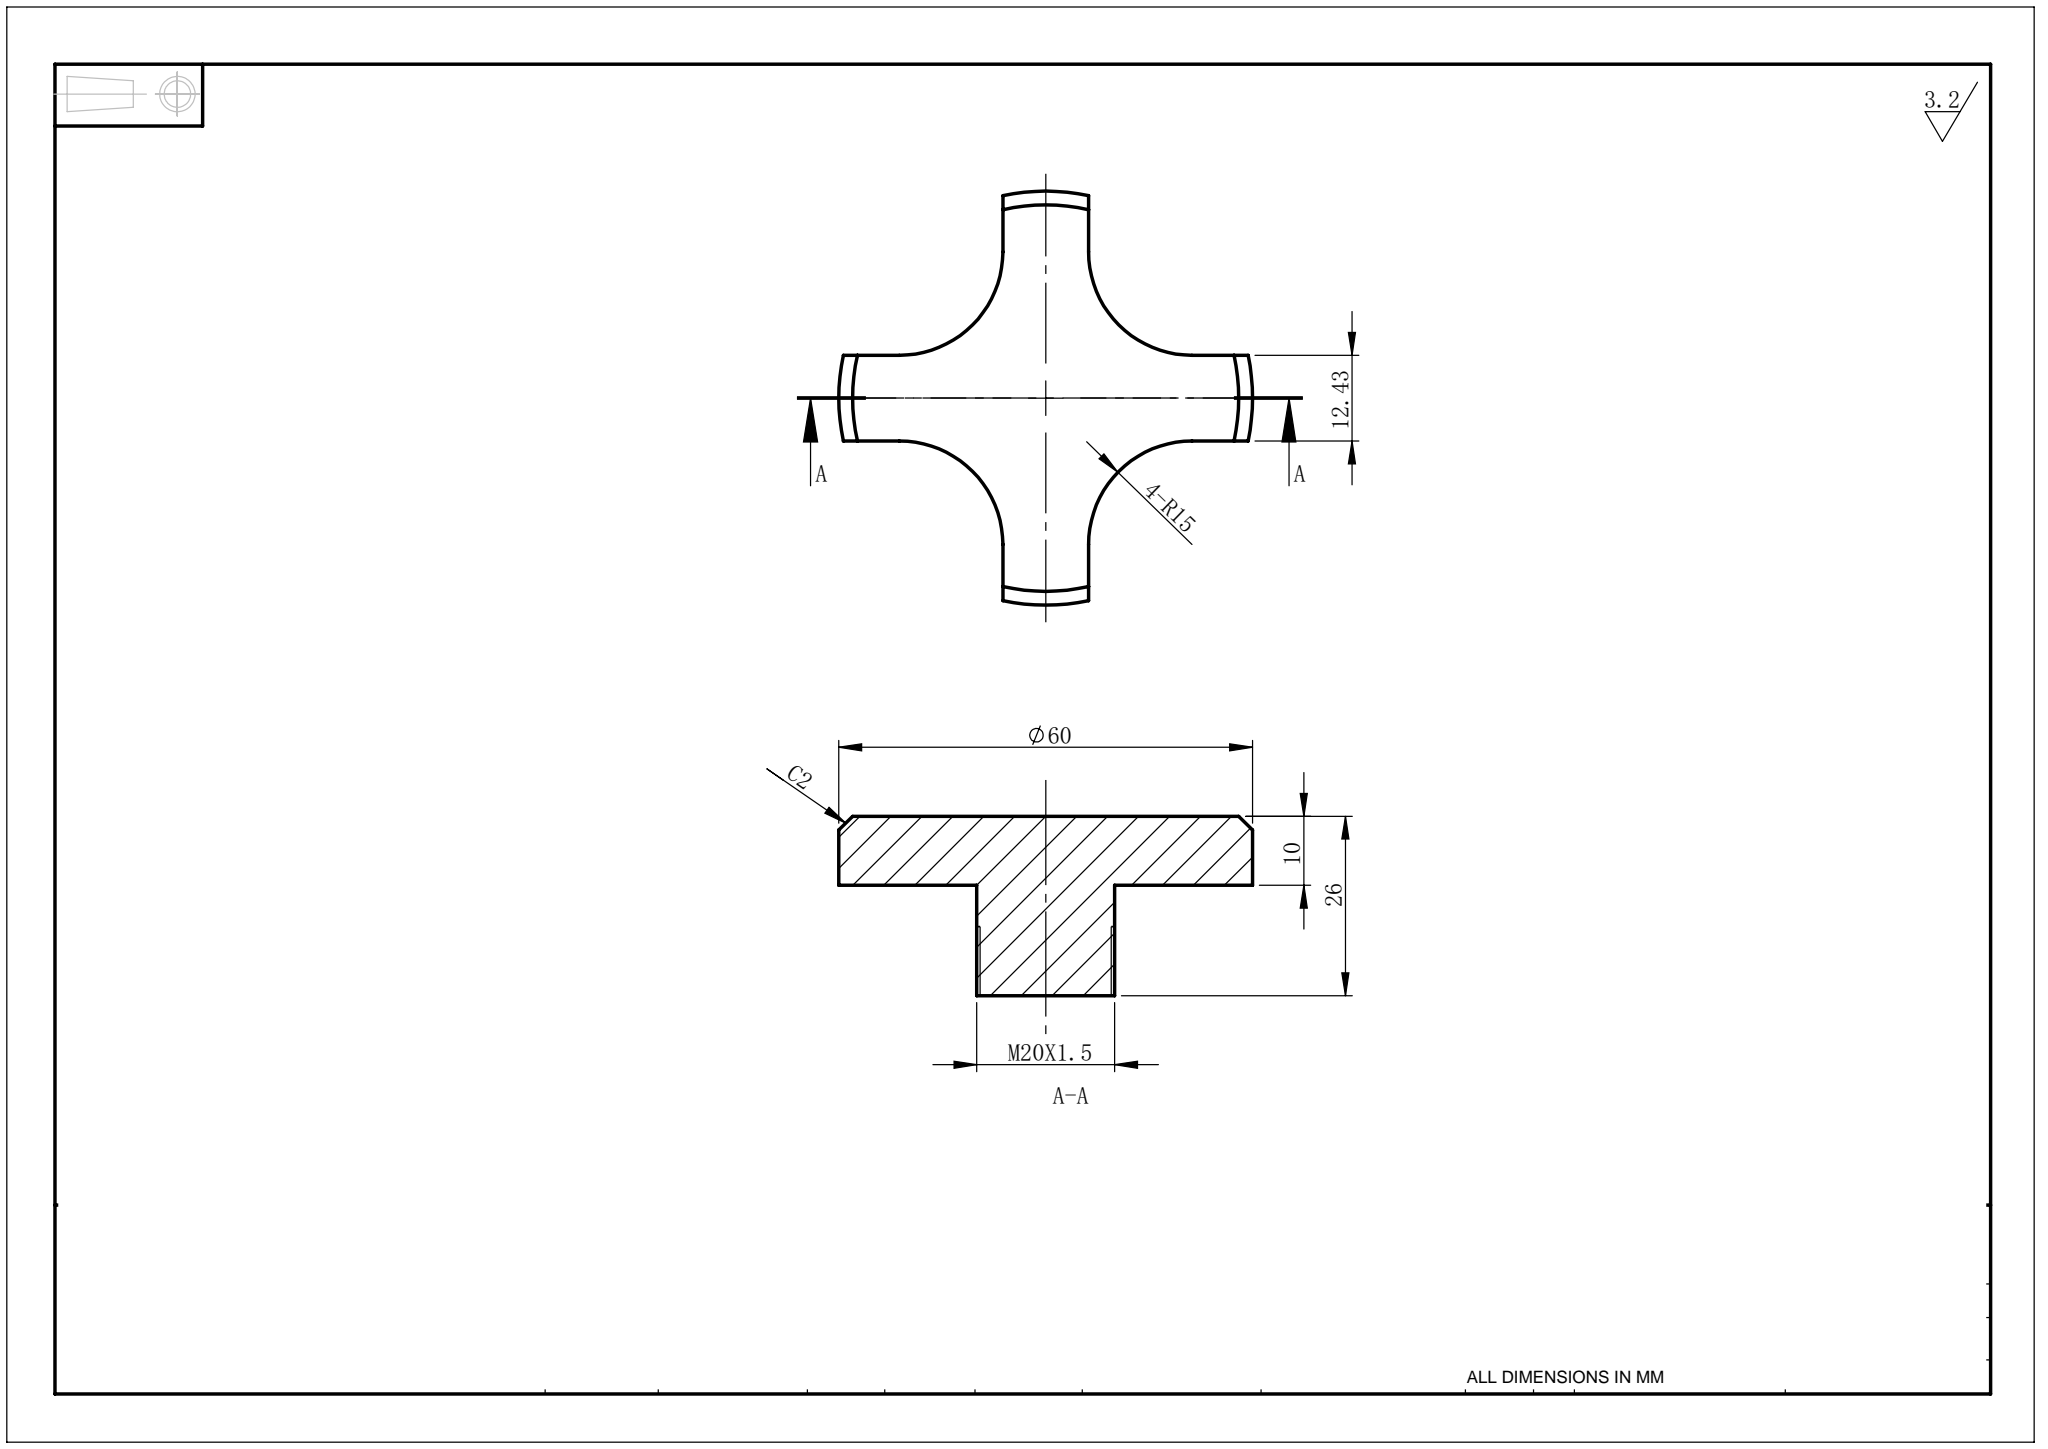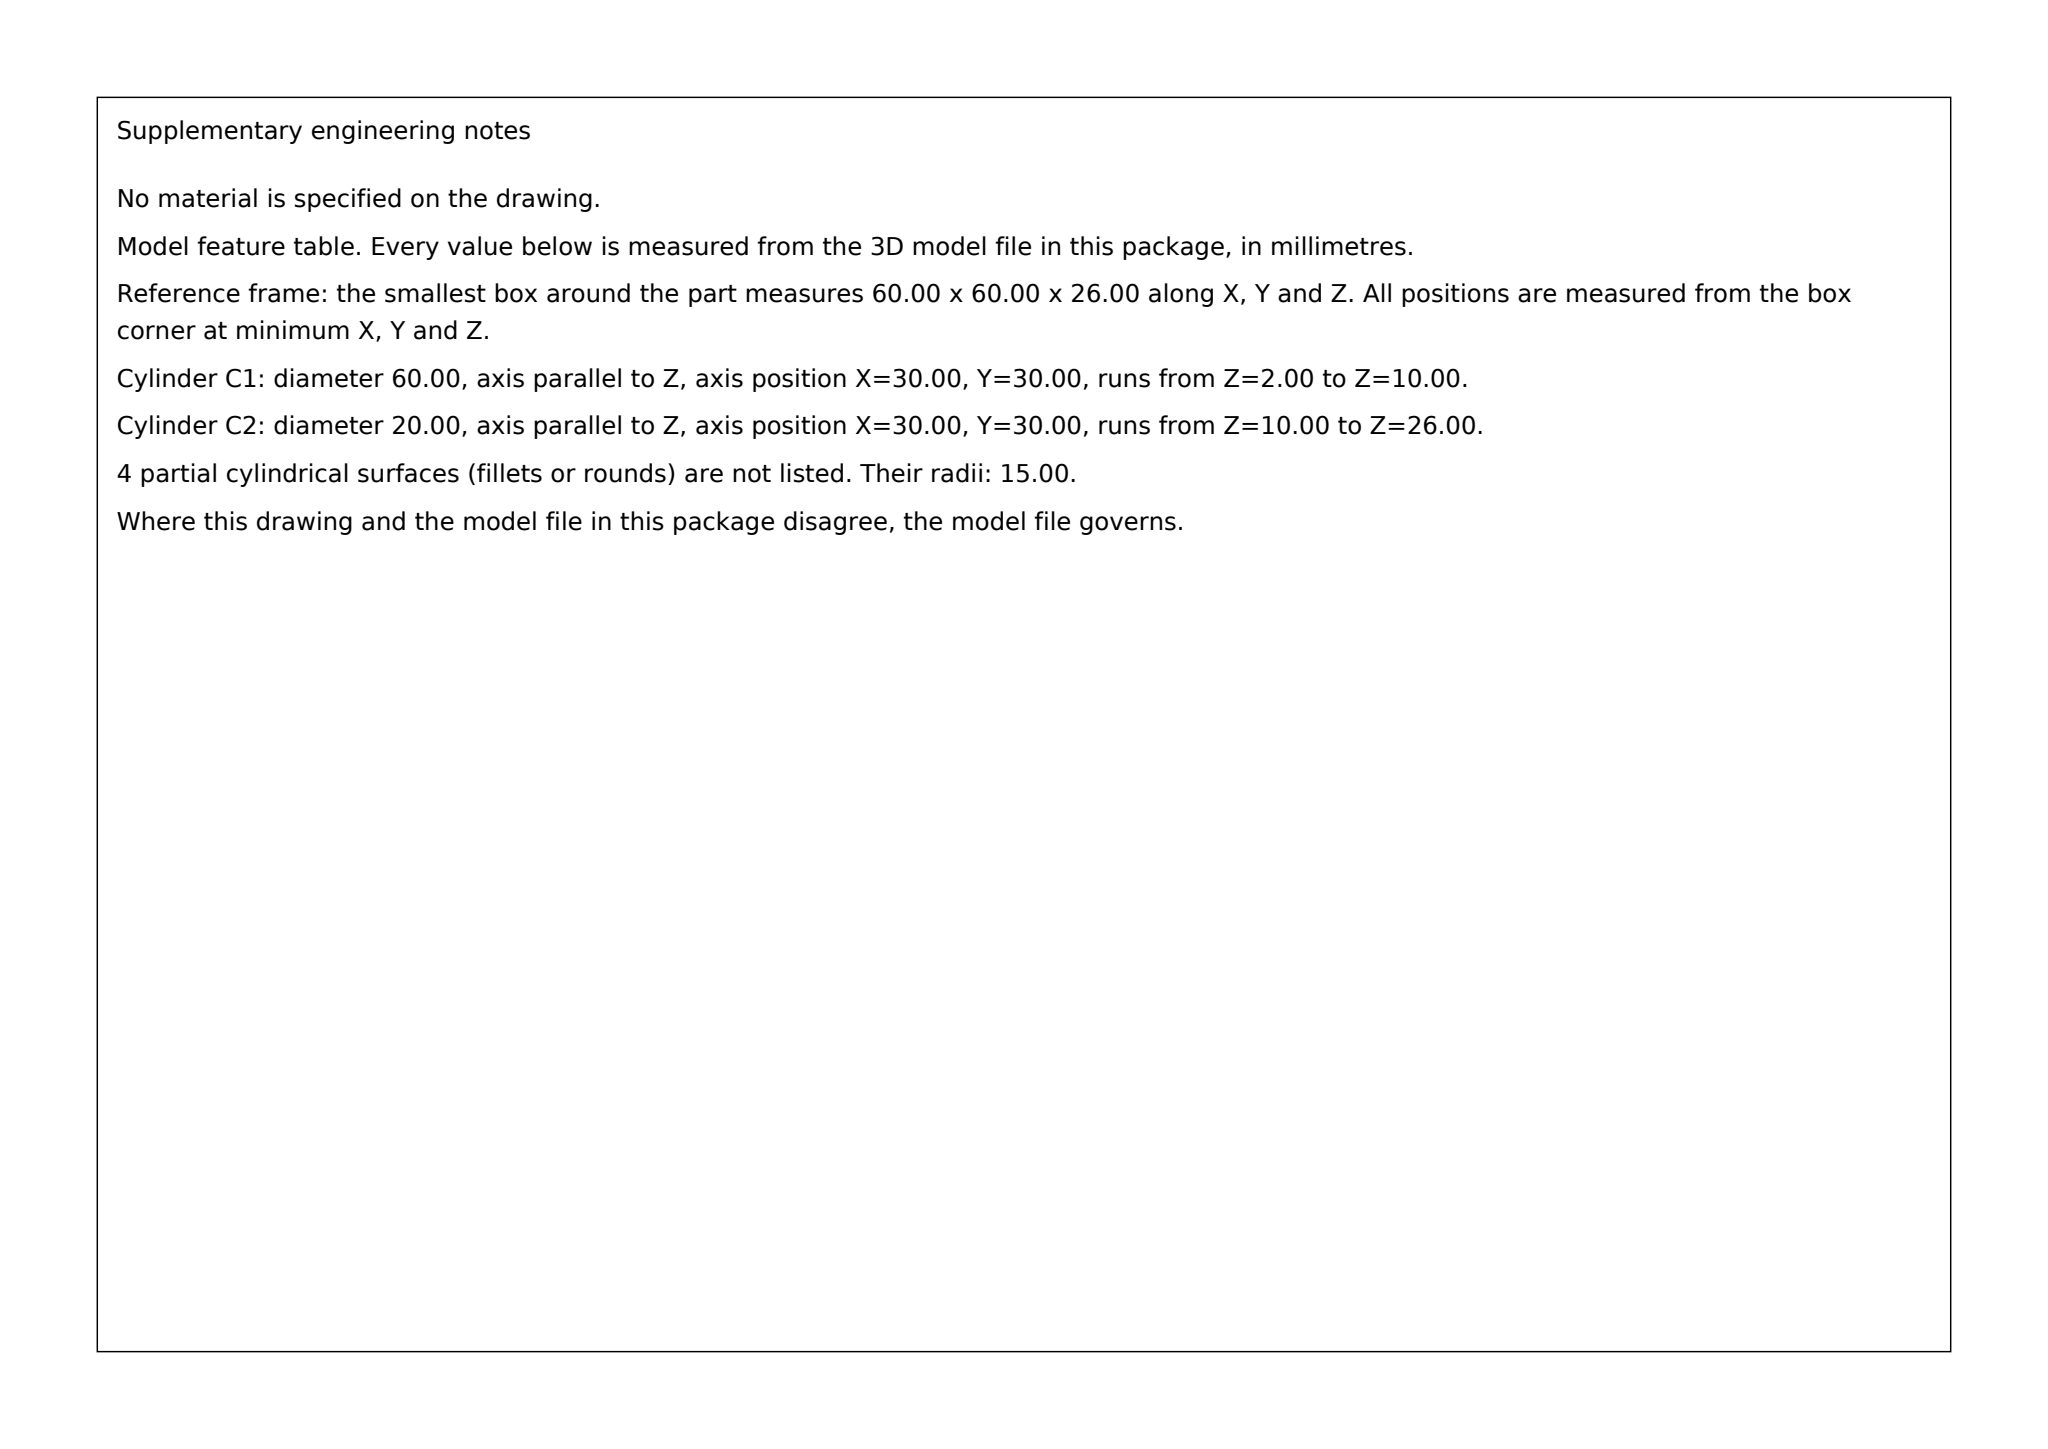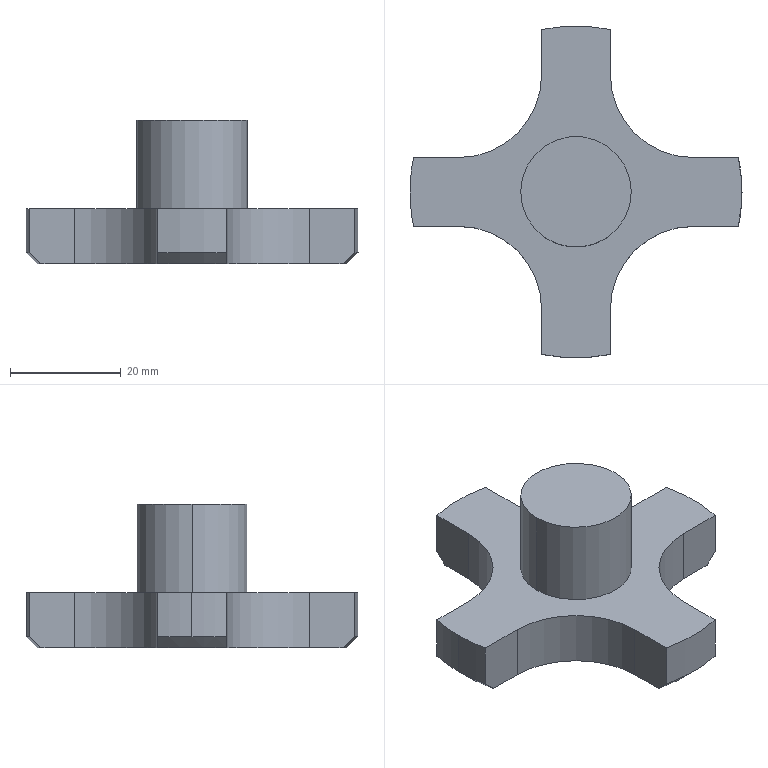Part | SolidWorks | mm | 1 solid | 27 faces | box 60 x 60 x 26 mm | volume 20118 mm3 | cylinder 11 | plane 11 | cone 5 | commonest cylinder face diameters 60 x5 30 x4 20 x2
build123d program:
from build123d import *

# Parameters (mm, degrees)
SKETCH1_R           = 30
BOSS_EXTRUDE1_DEPTH = 10
SKETCH2_R           = 10
BOSS_EXTRUDE2_DEPTH = 16
CUT_EXTRUDE1_DEPTH  = 16
CIRPATTERN1_COUNT   = 4
CHAMFER1_SIZE       = 2


with BuildPart() as part:
    # Sketch1 → Boss-Extrude1 (new body)
    with BuildSketch(Plane.XY):
        Circle(SKETCH1_R)
    extrude(amount=BOSS_EXTRUDE1_DEPTH)

    # Sketch2 → Boss-Extrude2 (add)
    with BuildSketch(Plane.XY.offset(10)):
        Circle(SKETCH2_R)
    extrude(amount=BOSS_EXTRUDE2_DEPTH)

    # Sketch3 → Cut-Extrude1 (cut)
    with BuildSketch(Plane(origin=(0, 0, 0), x_dir=(-1, 0, 0), z_dir=(0, 0, -1))):
        with BuildLine():
            Line((21.213, 6.213), (40.164, 6.213))
            Line((40.164, 6.213), (40.164, 40.733))
            Line((40.164, 40.733), (6.213, 40.733))
            Line((6.213, 40.733), (6.213, 21.213))
            ThreePointArc((6.213, 21.213), (10.607, 10.607), (21.213, 6.213))
        make_face()
    cut_extrude1 = extrude(amount=-CUT_EXTRUDE1_DEPTH, mode=Mode.SUBTRACT)

    # CirPattern1: Cut-Extrude1 ×4 about axis
    cirpattern1_axis = Axis((0, 0, 0), (0, 0, 1))
    for i in range(1, CIRPATTERN1_COUNT):
        add(cut_extrude1.rotate(cirpattern1_axis, i * 360 / CIRPATTERN1_COUNT), mode=Mode.SUBTRACT)

    # Chamfer1
    chamfer1_edges = [part.edges().sort_by_distance(p)[0] for p in [
        (-30, 0, 0),
        (0, 30, 0),
        (30, 0, 0),
        (0, -30, 0),
    ]]
    chamfer(chamfer1_edges, length=CHAMFER1_SIZE)


solid = part.part